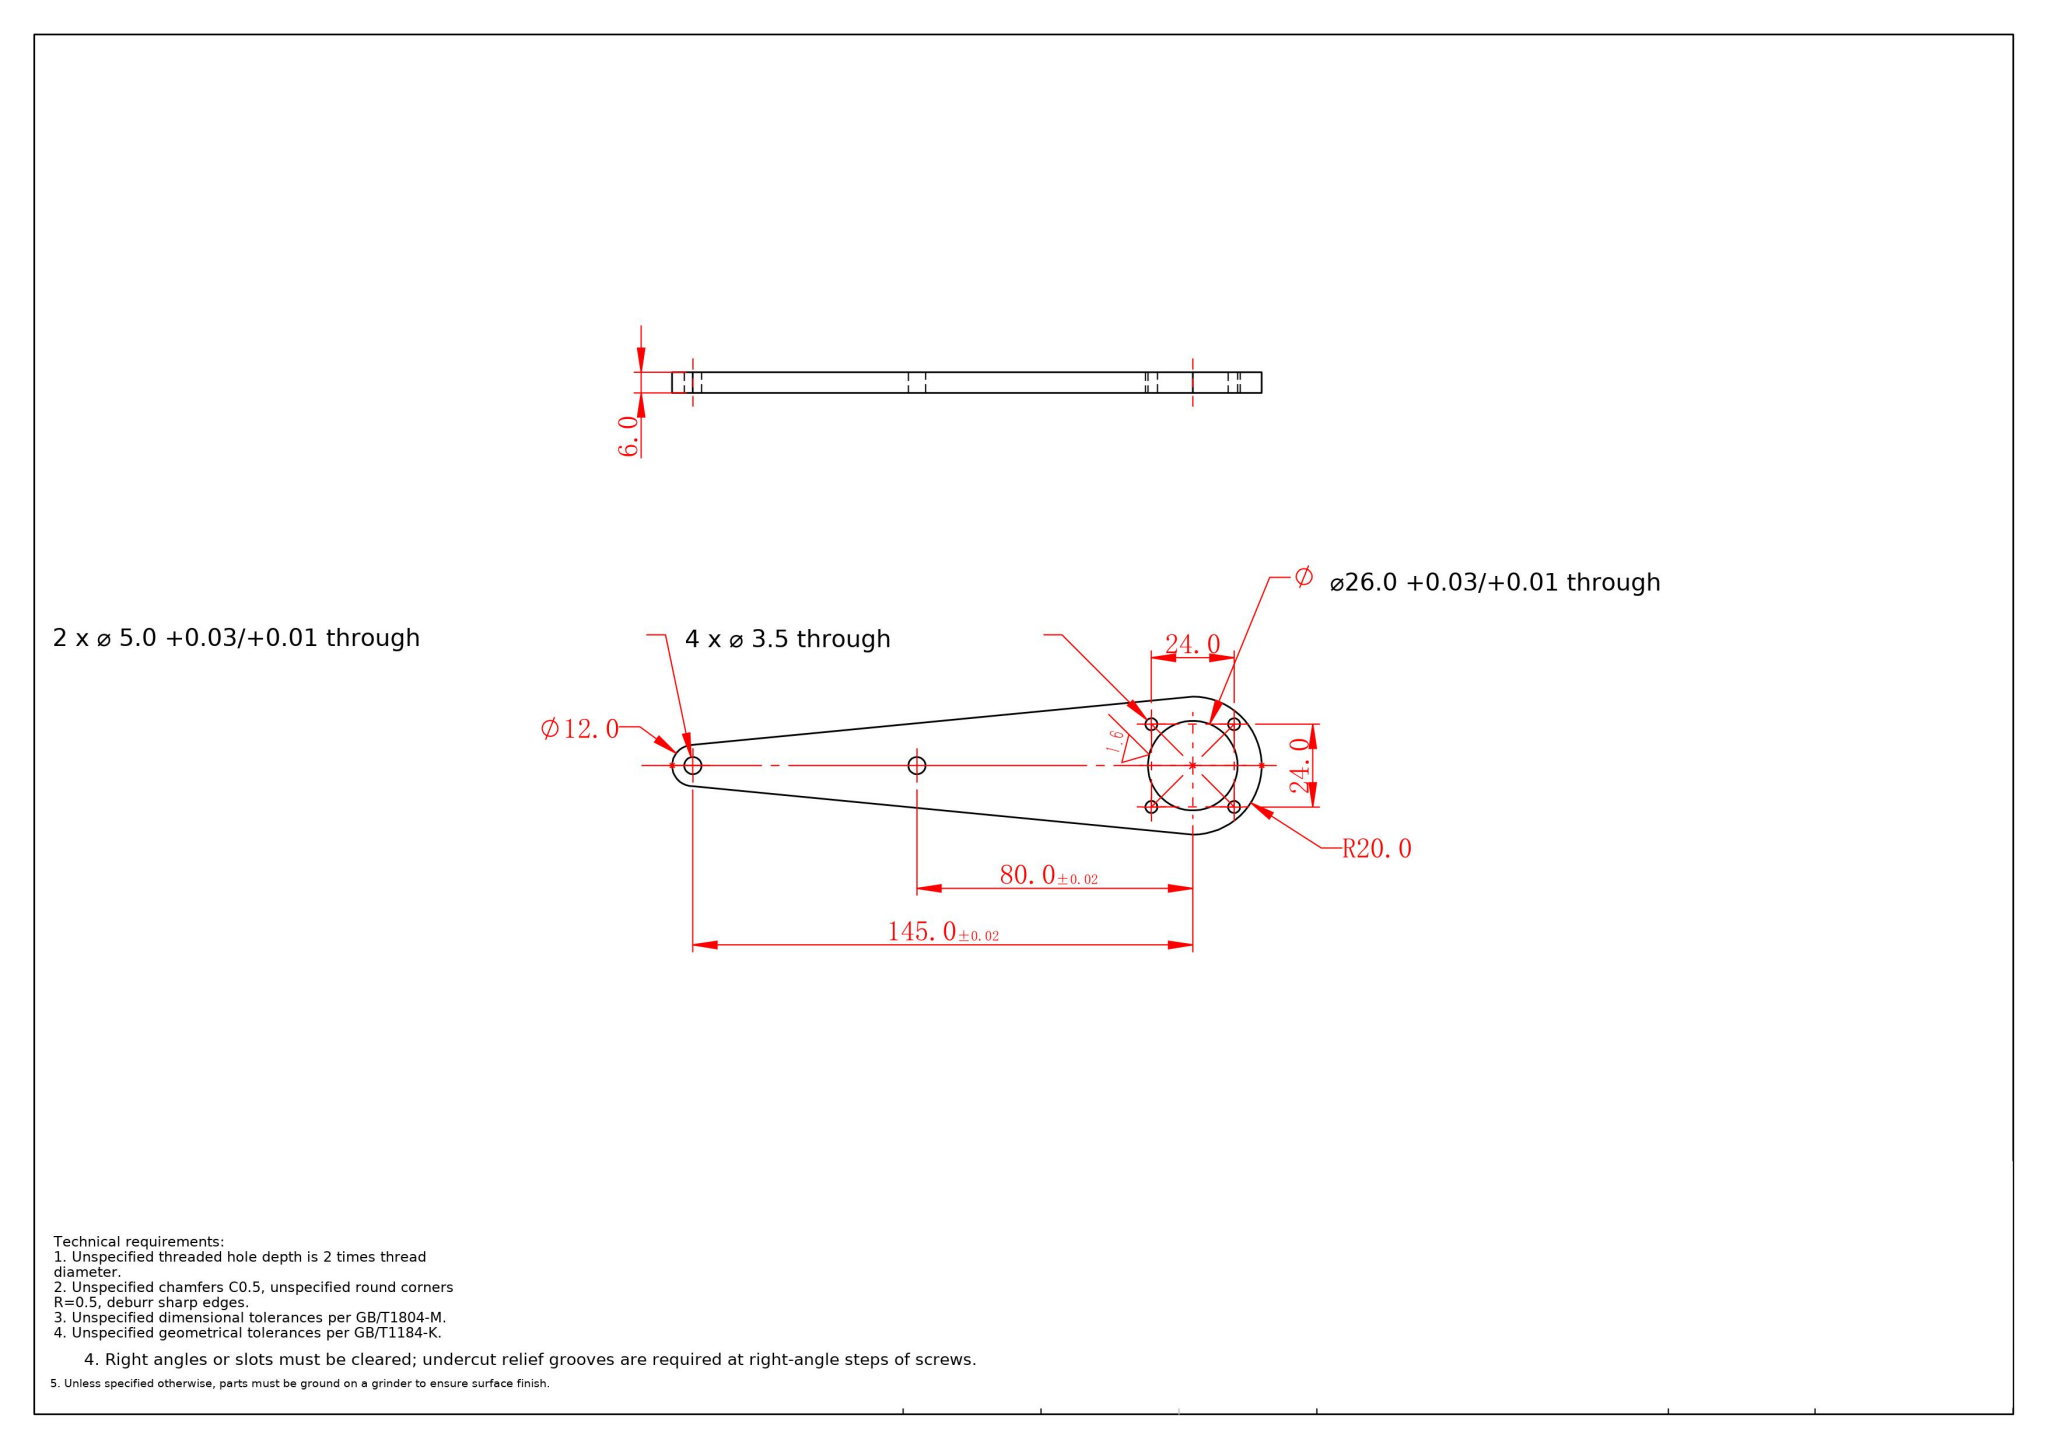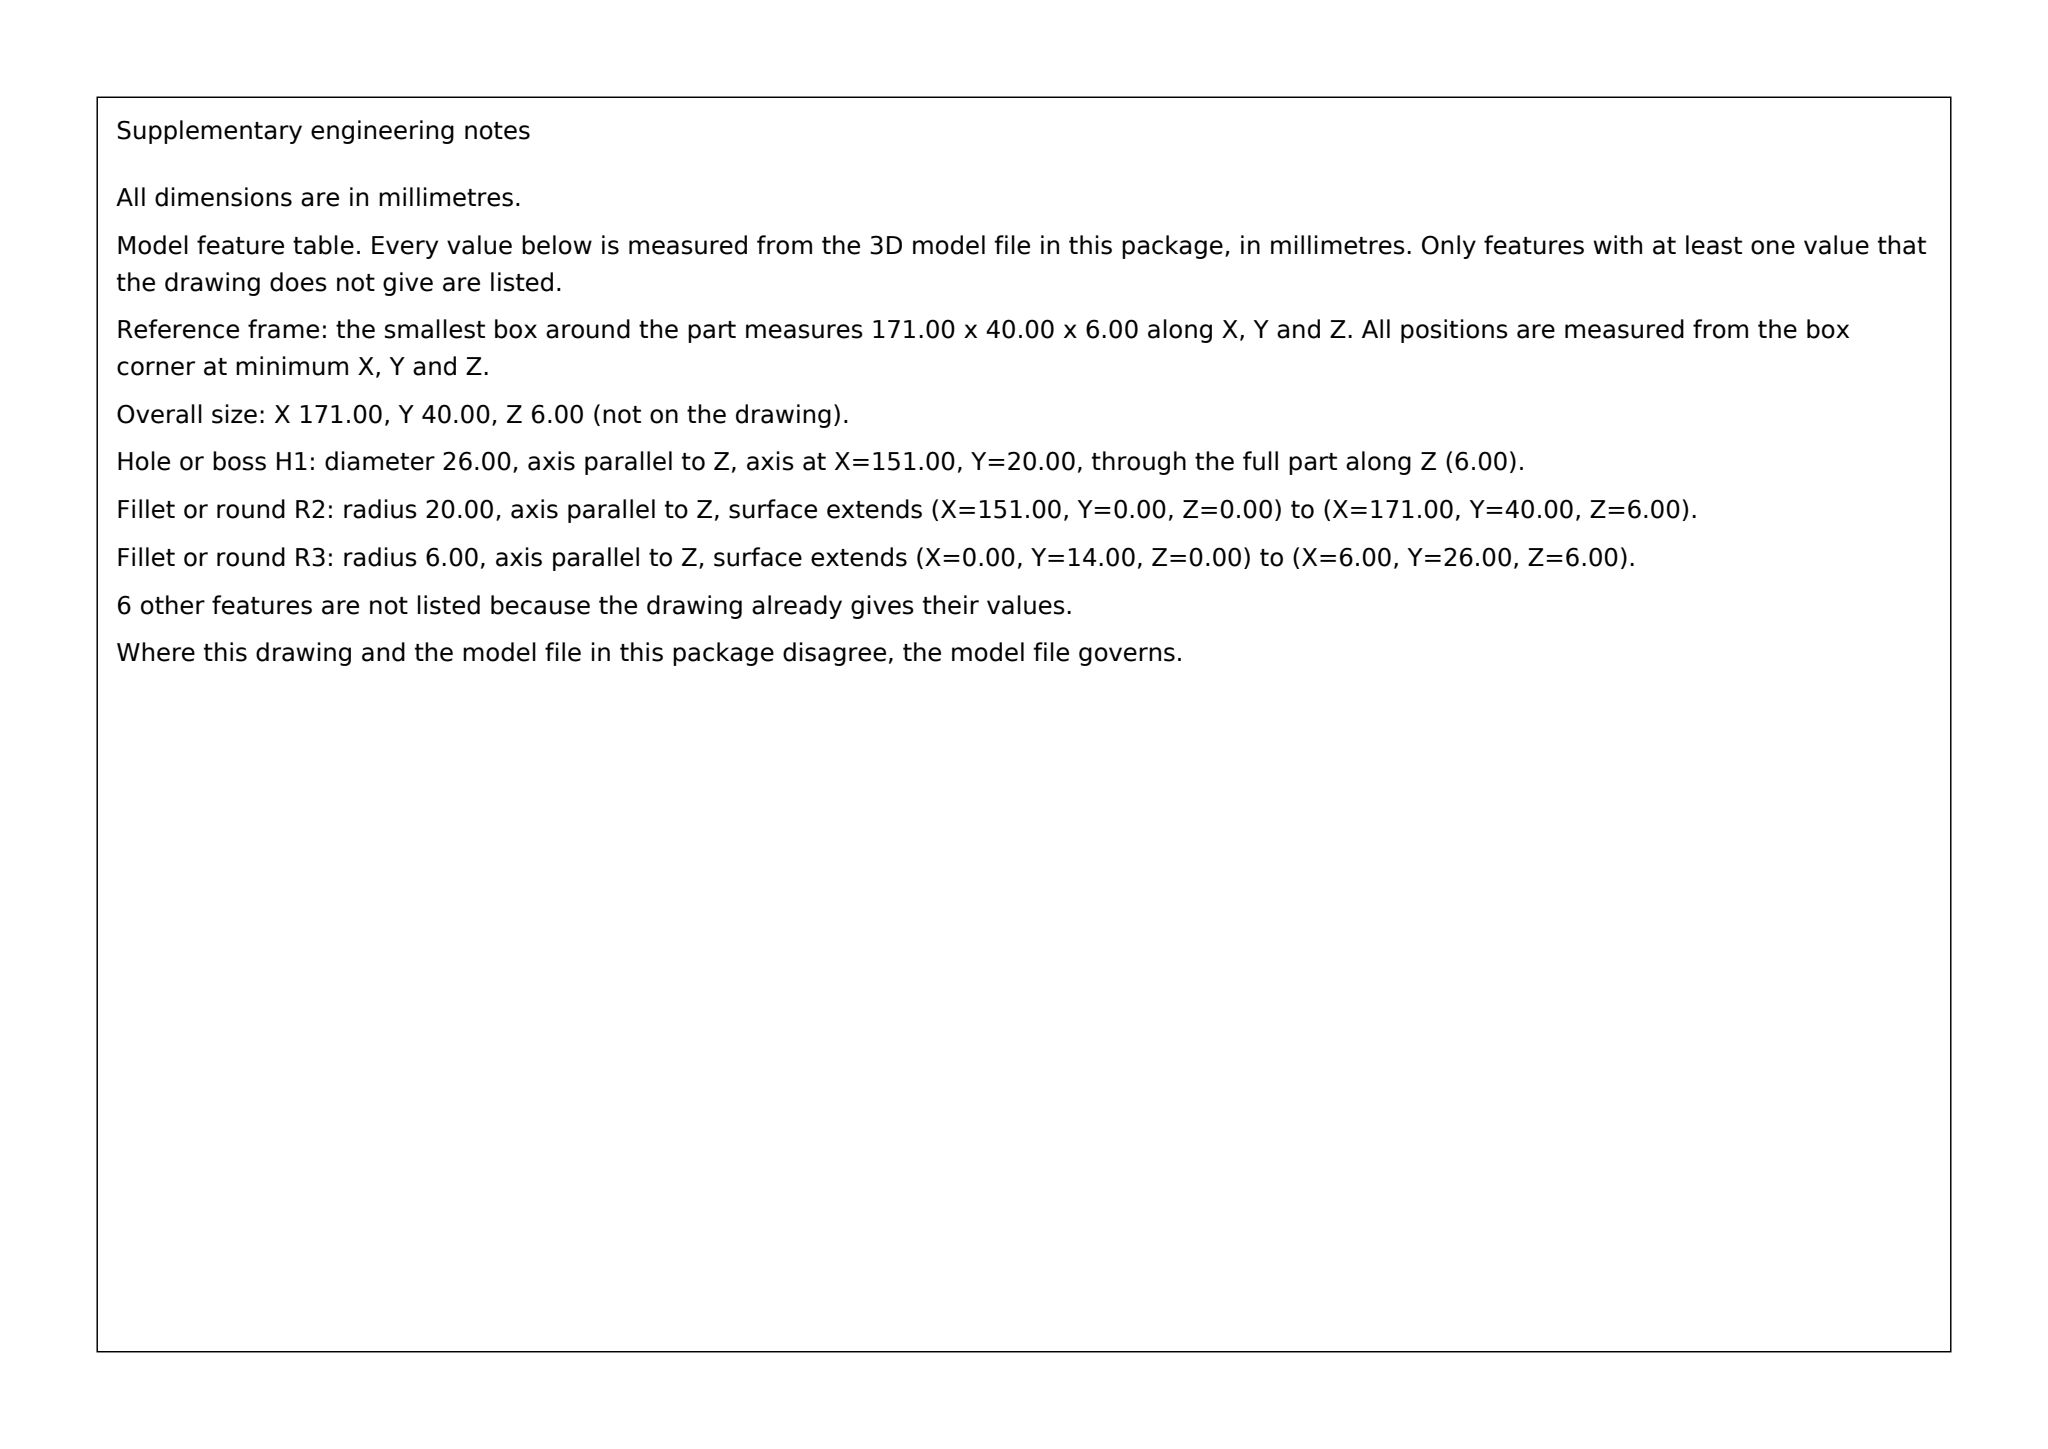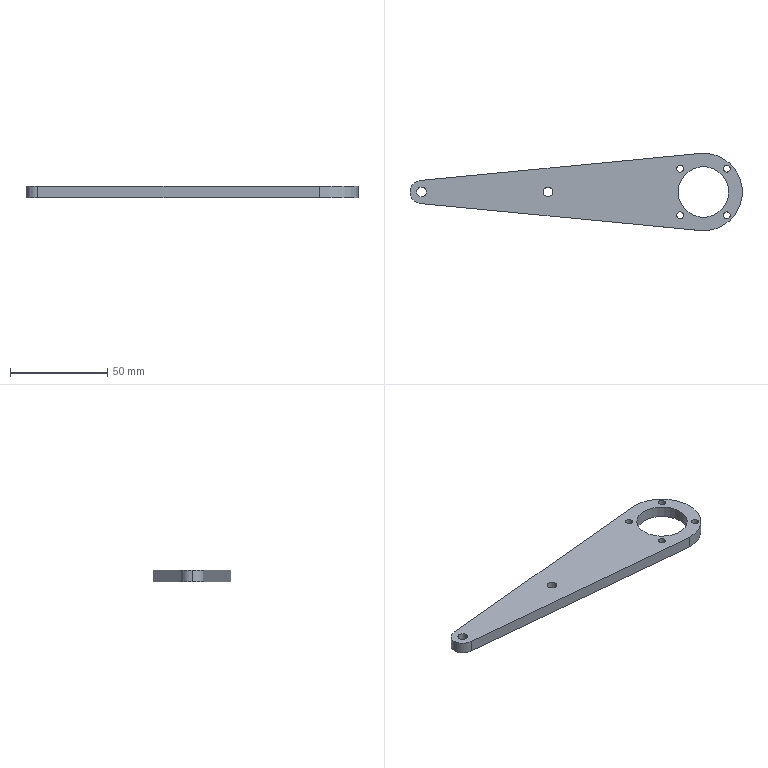Part | SolidWorks | mm | 1 solid | 21 faces | box 171 x 40 x 6 mm | volume 23077 mm3 | cylinder 17 | plane 4 | commonest cylinder face diameters 3.5 x8 5 x4 26 x2 12 x2 40 x1
build123d program:
from build123d import *

# Parameters (mm, degrees)
SKETCH1_R                      = 13
BOSS_EXTRUDE1_DEPTH            = 3
F_3_5_3_5_DIAMETER_HOLE1_D     = 3.5
F_3_5_3_5_DIAMETER_HOLE1_DEPTH = 6
F_5_0_5_DIAMETER_HOLE1_D       = 5


with BuildPart() as part:
    # Sketch1 → Boss-Extrude1 (new, symmetric)
    with BuildSketch(Plane.XY):
        with BuildLine():
            Line((-145, 6), (0, 20))
            ThreePointArc((0, 20), (20, 0), (0, -20))
            Line((0, -20), (-145, -6))
            ThreePointArc((-145, -6), (-151, 0), (-145, 6))
        make_face()
        Circle(SKETCH1_R, mode=Mode.SUBTRACT)
    extrude(amount=BOSS_EXTRUDE1_DEPTH, both=True)

    # 3.5 _3.5_ Diameter Hole1
    with Locations(Plane.XY.offset(3)):
        with Locations((0, 0), (12, -12), (-12, 12), (-12, -12), (12, 12)):
            Hole(F_3_5_3_5_DIAMETER_HOLE1_D / 2, depth=F_3_5_3_5_DIAMETER_HOLE1_DEPTH)

    # 5.0 _5_ Diameter Hole1 (through all)
    with Locations(Plane.XY.offset(3)):
        with Locations((-145, 0), (-80, 0)):
            Hole(F_5_0_5_DIAMETER_HOLE1_D / 2)


solid = part.part
STEP:
#1=CARTESIAN_POINT('',(-147.5,-0.,-3.));
#2=VERTEX_POINT('',#1);
#3=CARTESIAN_POINT('',(-142.5,-0.,-3.));
#4=VERTEX_POINT('',#3);
#5=CARTESIAN_POINT('',(-145.,-0.,-3.));
#6=DIRECTION('',(0.,0.,1.));
#7=DIRECTION('',(1.,0.,0.));
#8=AXIS2_PLACEMENT_3D('',#5,#6,#7);
#9=CIRCLE('',#8,2.5);
#10=EDGE_CURVE('',#2,#4,#9,.T.);
#11=ORIENTED_EDGE('',*,*,#10,.F.);
#12=CARTESIAN_POINT('',(-147.5,-0.,3.));
#13=VERTEX_POINT('',#12);
#14=CARTESIAN_POINT('',(-147.5,-0.,3.));
#15=DIRECTION('',(0.,0.,1.));
#16=VECTOR('',#15,1000.);
#17=LINE('',#14,#16);
#18=EDGE_CURVE('',#2,#13,#17,.T.);
#19=ORIENTED_EDGE('',*,*,#18,.T.);
#20=CARTESIAN_POINT('',(-142.5,-0.,3.));
#21=VERTEX_POINT('',#20);
#22=CARTESIAN_POINT('',(-145.,-0.,3.));
#23=DIRECTION('',(0.,0.,1.));
#24=DIRECTION('',(1.,0.,0.));
#25=AXIS2_PLACEMENT_3D('',#22,#23,#24);
#26=CIRCLE('',#25,2.5);
#27=EDGE_CURVE('',#13,#21,#26,.T.);
#28=ORIENTED_EDGE('',*,*,#27,.T.);
#29=CARTESIAN_POINT('',(-142.5,-0.,3.));
#30=DIRECTION('',(0.,0.,1.));
#31=VECTOR('',#30,1000.);
#32=LINE('',#29,#31);
#33=EDGE_CURVE('',#4,#21,#32,.T.);
#34=ORIENTED_EDGE('',*,*,#33,.F.);
#35=EDGE_LOOP('',(#11,#19,#28,#34));
#36=FACE_OUTER_BOUND('',#35,.T.);
#37=CARTESIAN_POINT('',(-145.,-0.,3.));
#38=DIRECTION('',(0.,0.,1.));
#39=DIRECTION('',(1.,0.,0.));
#40=AXIS2_PLACEMENT_3D('',#37,#38,#39);
#41=CYLINDRICAL_SURFACE('',#40,2.5);
#42=ADVANCED_FACE('',(#36),#41,.F.);
#43=CARTESIAN_POINT('',(-82.5,0.,-3.));
#44=VERTEX_POINT('',#43);
#45=CARTESIAN_POINT('',(-77.5,0.,-3.));
#46=VERTEX_POINT('',#45);
#47=CARTESIAN_POINT('',(-80.,0.,-3.));
#48=DIRECTION('',(0.,0.,1.));
#49=DIRECTION('',(1.,0.,0.));
#50=AXIS2_PLACEMENT_3D('',#47,#48,#49);
#51=CIRCLE('',#50,2.5);
#52=EDGE_CURVE('',#44,#46,#51,.T.);
#53=ORIENTED_EDGE('',*,*,#52,.F.);
#54=CARTESIAN_POINT('',(-82.5,0.,3.));
#55=VERTEX_POINT('',#54);
#56=CARTESIAN_POINT('',(-82.5,0.,3.));
#57=DIRECTION('',(0.,0.,1.));
#58=VECTOR('',#57,1000.);
#59=LINE('',#56,#58);
#60=EDGE_CURVE('',#44,#55,#59,.T.);
#61=ORIENTED_EDGE('',*,*,#60,.T.);
#62=CARTESIAN_POINT('',(-77.5,0.,3.));
#63=VERTEX_POINT('',#62);
#64=CARTESIAN_POINT('',(-80.,0.,3.));
#65=DIRECTION('',(0.,0.,1.));
#66=DIRECTION('',(1.,0.,0.));
#67=AXIS2_PLACEMENT_3D('',#64,#65,#66);
#68=CIRCLE('',#67,2.5);
#69=EDGE_CURVE('',#55,#63,#68,.T.);
#70=ORIENTED_EDGE('',*,*,#69,.T.);
#71=CARTESIAN_POINT('',(-77.5,0.,3.));
#72=DIRECTION('',(0.,0.,1.));
#73=VECTOR('',#72,1000.);
#74=LINE('',#71,#73);
#75=EDGE_CURVE('',#46,#63,#74,.T.);
#76=ORIENTED_EDGE('',*,*,#75,.F.);
#77=EDGE_LOOP('',(#53,#61,#70,#76));
#78=FACE_OUTER_BOUND('',#77,.T.);
#79=CARTESIAN_POINT('',(-80.,0.,3.));
#80=DIRECTION('',(0.,0.,1.));
#81=DIRECTION('',(1.,0.,0.));
#82=AXIS2_PLACEMENT_3D('',#79,#80,#81);
#83=CYLINDRICAL_SURFACE('',#82,2.5);
#84=ADVANCED_FACE('',(#78),#83,.F.);
#85=CARTESIAN_POINT('',(10.25,-12.,-3.));
#86=VERTEX_POINT('',#85);
#87=CARTESIAN_POINT('',(13.75,-12.,-3.));
#88=VERTEX_POINT('',#87);
#89=CARTESIAN_POINT('',(12.,-12.,-3.));
#90=DIRECTION('',(0.,0.,1.));
#91=DIRECTION('',(1.,0.,0.));
#92=AXIS2_PLACEMENT_3D('',#89,#90,#91);
#93=CIRCLE('',#92,1.75);
#94=EDGE_CURVE('',#86,#88,#93,.T.);
#95=ORIENTED_EDGE('',*,*,#94,.F.);
#96=CARTESIAN_POINT('',(10.25,-12.,3.));
#97=VERTEX_POINT('',#96);
#98=CARTESIAN_POINT('',(10.25,-12.,3.));
#99=DIRECTION('',(0.,0.,1.));
#100=VECTOR('',#99,1000.);
#101=LINE('',#98,#100);
#102=EDGE_CURVE('',#86,#97,#101,.T.);
#103=ORIENTED_EDGE('',*,*,#102,.T.);
#104=CARTESIAN_POINT('',(13.75,-12.,3.));
#105=VERTEX_POINT('',#104);
#106=CARTESIAN_POINT('',(12.,-12.,3.));
#107=DIRECTION('',(0.,0.,1.));
#108=DIRECTION('',(1.,0.,0.));
#109=AXIS2_PLACEMENT_3D('',#106,#107,#108);
#110=CIRCLE('',#109,1.75);
#111=EDGE_CURVE('',#97,#105,#110,.T.);
#112=ORIENTED_EDGE('',*,*,#111,.T.);
#113=CARTESIAN_POINT('',(13.75,-12.,3.));
#114=DIRECTION('',(0.,0.,1.));
#115=VECTOR('',#114,1000.);
#116=LINE('',#113,#115);
#117=EDGE_CURVE('',#88,#105,#116,.T.);
#118=ORIENTED_EDGE('',*,*,#117,.F.);
#119=EDGE_LOOP('',(#95,#103,#112,#118));
#120=FACE_OUTER_BOUND('',#119,.T.);
#121=CARTESIAN_POINT('',(12.,-12.,3.));
#122=DIRECTION('',(0.,0.,1.));
#123=DIRECTION('',(1.,0.,0.));
#124=AXIS2_PLACEMENT_3D('',#121,#122,#123);
#125=CYLINDRICAL_SURFACE('',#124,1.75);
#126=ADVANCED_FACE('',(#120),#125,.F.);
#127=CARTESIAN_POINT('',(-13.75,12.,-3.));
#128=VERTEX_POINT('',#127);
#129=CARTESIAN_POINT('',(-10.25,12.,-3.));
#130=VERTEX_POINT('',#129);
#131=CARTESIAN_POINT('',(-12.,12.,-3.));
#132=DIRECTION('',(0.,0.,1.));
#133=DIRECTION('',(1.,0.,0.));
#134=AXIS2_PLACEMENT_3D('',#131,#132,#133);
#135=CIRCLE('',#134,1.75);
#136=EDGE_CURVE('',#128,#130,#135,.T.);
#137=ORIENTED_EDGE('',*,*,#136,.F.);
#138=CARTESIAN_POINT('',(-13.75,12.,3.));
#139=VERTEX_POINT('',#138);
#140=CARTESIAN_POINT('',(-13.75,12.,3.));
#141=DIRECTION('',(0.,0.,1.));
#142=VECTOR('',#141,1000.);
#143=LINE('',#140,#142);
#144=EDGE_CURVE('',#128,#139,#143,.T.);
#145=ORIENTED_EDGE('',*,*,#144,.T.);
#146=CARTESIAN_POINT('',(-10.25,12.,3.));
#147=VERTEX_POINT('',#146);
#148=CARTESIAN_POINT('',(-12.,12.,3.));
#149=DIRECTION('',(0.,0.,1.));
#150=DIRECTION('',(1.,0.,0.));
#151=AXIS2_PLACEMENT_3D('',#148,#149,#150);
#152=CIRCLE('',#151,1.75);
#153=EDGE_CURVE('',#139,#147,#152,.T.);
#154=ORIENTED_EDGE('',*,*,#153,.T.);
#155=CARTESIAN_POINT('',(-10.25,12.,3.));
#156=DIRECTION('',(0.,0.,1.));
#157=VECTOR('',#156,1000.);
#158=LINE('',#155,#157);
#159=EDGE_CURVE('',#130,#147,#158,.T.);
#160=ORIENTED_EDGE('',*,*,#159,.F.);
#161=EDGE_LOOP('',(#137,#145,#154,#160));
#162=FACE_OUTER_BOUND('',#161,.T.);
#163=CARTESIAN_POINT('',(-12.,12.,3.));
#164=DIRECTION('',(0.,0.,1.));
#165=DIRECTION('',(1.,0.,0.));
#166=AXIS2_PLACEMENT_3D('',#163,#164,#165);
#167=CYLINDRICAL_SURFACE('',#166,1.75);
#168=ADVANCED_FACE('',(#162),#167,.F.);
#169=CARTESIAN_POINT('',(-13.75,-12.,-3.));
#170=VERTEX_POINT('',#169);
#171=CARTESIAN_POINT('',(-10.25,-12.,-3.));
#172=VERTEX_POINT('',#171);
#173=CARTESIAN_POINT('',(-12.,-12.,-3.));
#174=DIRECTION('',(0.,0.,1.));
#175=DIRECTION('',(1.,0.,0.));
#176=AXIS2_PLACEMENT_3D('',#173,#174,#175);
#177=CIRCLE('',#176,1.75);
#178=EDGE_CURVE('',#170,#172,#177,.T.);
#179=ORIENTED_EDGE('',*,*,#178,.F.);
#180=CARTESIAN_POINT('',(-13.75,-12.,3.));
#181=VERTEX_POINT('',#180);
#182=CARTESIAN_POINT('',(-13.75,-12.,3.));
#183=DIRECTION('',(0.,0.,1.));
#184=VECTOR('',#183,1000.);
#185=LINE('',#182,#184);
#186=EDGE_CURVE('',#170,#181,#185,.T.);
#187=ORIENTED_EDGE('',*,*,#186,.T.);
#188=CARTESIAN_POINT('',(-10.25,-12.,3.));
#189=VERTEX_POINT('',#188);
#190=CARTESIAN_POINT('',(-12.,-12.,3.));
#191=DIRECTION('',(0.,0.,1.));
#192=DIRECTION('',(1.,0.,0.));
#193=AXIS2_PLACEMENT_3D('',#190,#191,#192);
#194=CIRCLE('',#193,1.75);
#195=EDGE_CURVE('',#181,#189,#194,.T.);
#196=ORIENTED_EDGE('',*,*,#195,.T.);
#197=CARTESIAN_POINT('',(-10.25,-12.,3.));
#198=DIRECTION('',(0.,0.,1.));
#199=VECTOR('',#198,1000.);
#200=LINE('',#197,#199);
#201=EDGE_CURVE('',#172,#189,#200,.T.);
#202=ORIENTED_EDGE('',*,*,#201,.F.);
#203=EDGE_LOOP('',(#179,#187,#196,#202));
#204=FACE_OUTER_BOUND('',#203,.T.);
#205=CARTESIAN_POINT('',(-12.,-12.,3.));
#206=DIRECTION('',(0.,0.,1.));
#207=DIRECTION('',(1.,0.,0.));
#208=AXIS2_PLACEMENT_3D('',#205,#206,#207);
#209=CYLINDRICAL_SURFACE('',#208,1.75);
#210=ADVANCED_FACE('',(#204),#209,.F.);
#211=CARTESIAN_POINT('',(10.25,12.,-3.));
#212=VERTEX_POINT('',#211);
#213=CARTESIAN_POINT('',(13.75,12.,-3.));
#214=VERTEX_POINT('',#213);
#215=CARTESIAN_POINT('',(12.,12.,-3.));
#216=DIRECTION('',(0.,0.,1.));
#217=DIRECTION('',(1.,0.,0.));
#218=AXIS2_PLACEMENT_3D('',#215,#216,#217);
#219=CIRCLE('',#218,1.75);
#220=EDGE_CURVE('',#212,#214,#219,.T.);
#221=ORIENTED_EDGE('',*,*,#220,.F.);
#222=CARTESIAN_POINT('',(10.25,12.,3.));
#223=VERTEX_POINT('',#222);
#224=CARTESIAN_POINT('',(10.25,12.,3.));
#225=DIRECTION('',(0.,0.,1.));
#226=VECTOR('',#225,1000.);
#227=LINE('',#224,#226);
#228=EDGE_CURVE('',#212,#223,#227,.T.);
#229=ORIENTED_EDGE('',*,*,#228,.T.);
#230=CARTESIAN_POINT('',(13.75,12.,3.));
#231=VERTEX_POINT('',#230);
#232=CARTESIAN_POINT('',(12.,12.,3.));
#233=DIRECTION('',(0.,0.,1.));
#234=DIRECTION('',(1.,0.,0.));
#235=AXIS2_PLACEMENT_3D('',#232,#233,#234);
#236=CIRCLE('',#235,1.75);
#237=EDGE_CURVE('',#223,#231,#236,.T.);
#238=ORIENTED_EDGE('',*,*,#237,.T.);
#239=CARTESIAN_POINT('',(13.75,12.,3.));
#240=DIRECTION('',(0.,0.,1.));
#241=VECTOR('',#240,1000.);
#242=LINE('',#239,#241);
#243=EDGE_CURVE('',#214,#231,#242,.T.);
#244=ORIENTED_EDGE('',*,*,#243,.F.);
#245=EDGE_LOOP('',(#221,#229,#238,#244));
#246=FACE_OUTER_BOUND('',#245,.T.);
#247=CARTESIAN_POINT('',(12.,12.,3.));
#248=DIRECTION('',(0.,0.,1.));
#249=DIRECTION('',(1.,0.,0.));
#250=AXIS2_PLACEMENT_3D('',#247,#248,#249);
#251=CYLINDRICAL_SURFACE('',#250,1.75);
#252=ADVANCED_FACE('',(#246),#251,.F.);
#253=CARTESIAN_POINT('',(-13.,0.,3.));
#254=VERTEX_POINT('',#253);
#255=CARTESIAN_POINT('',(13.,0.,3.));
#256=VERTEX_POINT('',#255);
#257=CARTESIAN_POINT('',(0.,0.,3.));
#258=DIRECTION('',(0.,0.,1.));
#259=DIRECTION('',(1.,0.,0.));
#260=AXIS2_PLACEMENT_3D('',#257,#258,#259);
#261=CIRCLE('',#260,13.);
#262=EDGE_CURVE('',#254,#256,#261,.T.);
#263=ORIENTED_EDGE('',*,*,#262,.T.);
#264=CARTESIAN_POINT('',(13.,0.,-3.));
#265=VERTEX_POINT('',#264);
#266=CARTESIAN_POINT('',(13.,0.,3.));
#267=DIRECTION('',(0.,0.,-1.));
#268=VECTOR('',#267,1000.);
#269=LINE('',#266,#268);
#270=EDGE_CURVE('',#256,#265,#269,.T.);
#271=ORIENTED_EDGE('',*,*,#270,.T.);
#272=CARTESIAN_POINT('',(-13.,0.,-3.));
#273=VERTEX_POINT('',#272);
#274=CARTESIAN_POINT('',(0.,0.,-3.));
#275=DIRECTION('',(0.,0.,1.));
#276=DIRECTION('',(1.,0.,0.));
#277=AXIS2_PLACEMENT_3D('',#274,#275,#276);
#278=CIRCLE('',#277,13.);
#279=EDGE_CURVE('',#273,#265,#278,.T.);
#280=ORIENTED_EDGE('',*,*,#279,.F.);
#281=CARTESIAN_POINT('',(-13.,0.,3.));
#282=DIRECTION('',(0.,0.,-1.));
#283=VECTOR('',#282,1000.);
#284=LINE('',#281,#283);
#285=EDGE_CURVE('',#254,#273,#284,.T.);
#286=ORIENTED_EDGE('',*,*,#285,.F.);
#287=EDGE_LOOP('',(#263,#271,#280,#286));
#288=FACE_OUTER_BOUND('',#287,.T.);
#289=CARTESIAN_POINT('',(0.,0.,3.));
#290=DIRECTION('',(0.,0.,-1.));
#291=DIRECTION('',(-1.,0.,0.));
#292=AXIS2_PLACEMENT_3D('',#289,#290,#291);
#293=CYLINDRICAL_SURFACE('',#292,13.);
#294=ADVANCED_FACE('',(#288),#293,.F.);
#295=CARTESIAN_POINT('',(-151.,-0.,3.));
#296=VERTEX_POINT('',#295);
#297=CARTESIAN_POINT('',(-145.,-6.,3.));
#298=VERTEX_POINT('',#297);
#299=CARTESIAN_POINT('',(-145.,-0.,3.));
#300=DIRECTION('',(0.,0.,1.));
#301=DIRECTION('',(1.,0.,0.));
#302=AXIS2_PLACEMENT_3D('',#299,#300,#301);
#303=CIRCLE('',#302,6.);
#304=EDGE_CURVE('',#296,#298,#303,.T.);
#305=ORIENTED_EDGE('',*,*,#304,.F.);
#306=CARTESIAN_POINT('',(-151.,-0.,-3.));
#307=VERTEX_POINT('',#306);
#308=CARTESIAN_POINT('',(-151.,-0.,3.));
#309=DIRECTION('',(0.,0.,-1.));
#310=VECTOR('',#309,1000.);
#311=LINE('',#308,#310);
#312=EDGE_CURVE('',#296,#307,#311,.T.);
#313=ORIENTED_EDGE('',*,*,#312,.T.);
#314=CARTESIAN_POINT('',(-145.,-6.,-3.));
#315=VERTEX_POINT('',#314);
#316=CARTESIAN_POINT('',(-145.,-0.,-3.));
#317=DIRECTION('',(0.,0.,1.));
#318=DIRECTION('',(1.,0.,0.));
#319=AXIS2_PLACEMENT_3D('',#316,#317,#318);
#320=CIRCLE('',#319,6.);
#321=EDGE_CURVE('',#307,#315,#320,.T.);
#322=ORIENTED_EDGE('',*,*,#321,.T.);
#323=CARTESIAN_POINT('',(-145.,-6.,3.));
#324=DIRECTION('',(0.,0.,-1.));
#325=VECTOR('',#324,1000.);
#326=LINE('',#323,#325);
#327=EDGE_CURVE('',#298,#315,#326,.T.);
#328=ORIENTED_EDGE('',*,*,#327,.F.);
#329=EDGE_LOOP('',(#305,#313,#322,#328));
#330=FACE_OUTER_BOUND('',#329,.T.);
#331=CARTESIAN_POINT('',(-145.,-0.,3.));
#332=DIRECTION('',(0.,0.,-1.));
#333=DIRECTION('',(-1.,0.,0.));
#334=AXIS2_PLACEMENT_3D('',#331,#332,#333);
#335=CYLINDRICAL_SURFACE('',#334,6.);
#336=ADVANCED_FACE('',(#330),#335,.T.);
#337=CARTESIAN_POINT('',(-145.,-0.,3.));
#338=DIRECTION('',(0.,0.,1.));
#339=DIRECTION('',(1.,0.,0.));
#340=AXIS2_PLACEMENT_3D('',#337,#338,#339);
#341=CIRCLE('',#340,2.5);
#342=EDGE_CURVE('',#21,#13,#341,.T.);
#343=ORIENTED_EDGE('',*,*,#342,.F.);
#344=ORIENTED_EDGE('',*,*,#27,.F.);
#345=EDGE_LOOP('',(#343,#344));
#346=FACE_BOUND('',#345,.T.);
#347=CARTESIAN_POINT('',(-80.,0.,3.));
#348=DIRECTION('',(0.,0.,1.));
#349=DIRECTION('',(1.,0.,0.));
#350=AXIS2_PLACEMENT_3D('',#347,#348,#349);
#351=CIRCLE('',#350,2.5);
#352=EDGE_CURVE('',#63,#55,#351,.T.);
#353=ORIENTED_EDGE('',*,*,#352,.F.);
#354=ORIENTED_EDGE('',*,*,#69,.F.);
#355=EDGE_LOOP('',(#353,#354));
#356=FACE_BOUND('',#355,.T.);
#357=CARTESIAN_POINT('',(12.,-12.,3.));
#358=DIRECTION('',(0.,0.,1.));
#359=DIRECTION('',(1.,0.,0.));
#360=AXIS2_PLACEMENT_3D('',#357,#358,#359);
#361=CIRCLE('',#360,1.75);
#362=EDGE_CURVE('',#105,#97,#361,.T.);
#363=ORIENTED_EDGE('',*,*,#362,.F.);
#364=ORIENTED_EDGE('',*,*,#111,.F.);
#365=EDGE_LOOP('',(#363,#364));
#366=FACE_BOUND('',#365,.T.);
#367=CARTESIAN_POINT('',(-12.,12.,3.));
#368=DIRECTION('',(0.,0.,1.));
#369=DIRECTION('',(1.,0.,0.));
#370=AXIS2_PLACEMENT_3D('',#367,#368,#369);
#371=CIRCLE('',#370,1.75);
#372=EDGE_CURVE('',#147,#139,#371,.T.);
#373=ORIENTED_EDGE('',*,*,#372,.F.);
#374=ORIENTED_EDGE('',*,*,#153,.F.);
#375=EDGE_LOOP('',(#373,#374));
#376=FACE_BOUND('',#375,.T.);
#377=CARTESIAN_POINT('',(-12.,-12.,3.));
#378=DIRECTION('',(0.,0.,1.));
#379=DIRECTION('',(1.,0.,0.));
#380=AXIS2_PLACEMENT_3D('',#377,#378,#379);
#381=CIRCLE('',#380,1.75);
#382=EDGE_CURVE('',#189,#181,#381,.T.);
#383=ORIENTED_EDGE('',*,*,#382,.F.);
#384=ORIENTED_EDGE('',*,*,#195,.F.);
#385=EDGE_LOOP('',(#383,#384));
#386=FACE_BOUND('',#385,.T.);
#387=CARTESIAN_POINT('',(12.,12.,3.));
#388=DIRECTION('',(0.,0.,1.));
#389=DIRECTION('',(1.,0.,0.));
#390=AXIS2_PLACEMENT_3D('',#387,#388,#389);
#391=CIRCLE('',#390,1.75);
#392=EDGE_CURVE('',#231,#223,#391,.T.);
#393=ORIENTED_EDGE('',*,*,#392,.F.);
#394=ORIENTED_EDGE('',*,*,#237,.F.);
#395=EDGE_LOOP('',(#393,#394));
#396=FACE_BOUND('',#395,.T.);
#397=CARTESIAN_POINT('',(0.,-20.,3.));
#398=VERTEX_POINT('',#397);
#399=CARTESIAN_POINT('',(0.,20.,3.));
#400=VERTEX_POINT('',#399);
#401=CARTESIAN_POINT('',(0.,0.,3.));
#402=DIRECTION('',(0.,0.,1.));
#403=DIRECTION('',(1.,0.,0.));
#404=AXIS2_PLACEMENT_3D('',#401,#402,#403);
#405=CIRCLE('',#404,20.);
#406=EDGE_CURVE('',#398,#400,#405,.T.);
#407=ORIENTED_EDGE('',*,*,#406,.T.);
#408=CARTESIAN_POINT('',(-145.,6.,3.));
#409=VERTEX_POINT('',#408);
#410=CARTESIAN_POINT('',(-145.,6.,3.));
#411=DIRECTION('',(-0.9954,-0.0961,0.));
#412=VECTOR('',#411,1000.);
#413=LINE('',#410,#412);
#414=EDGE_CURVE('',#400,#409,#413,.T.);
#415=ORIENTED_EDGE('',*,*,#414,.T.);
#416=CARTESIAN_POINT('',(-145.,-0.,3.));
#417=DIRECTION('',(0.,0.,1.));
#418=DIRECTION('',(1.,0.,0.));
#419=AXIS2_PLACEMENT_3D('',#416,#417,#418);
#420=CIRCLE('',#419,6.);
#421=EDGE_CURVE('',#409,#296,#420,.T.);
#422=ORIENTED_EDGE('',*,*,#421,.T.);
#423=ORIENTED_EDGE('',*,*,#304,.T.);
#424=CARTESIAN_POINT('',(-145.,-6.,3.));
#425=DIRECTION('',(0.9954,-0.0961,0.));
#426=VECTOR('',#425,1000.);
#427=LINE('',#424,#426);
#428=EDGE_CURVE('',#298,#398,#427,.T.);
#429=ORIENTED_EDGE('',*,*,#428,.T.);
#430=EDGE_LOOP('',(#407,#415,#422,#423,#429));
#431=FACE_OUTER_BOUND('',#430,.T.);
#432=ORIENTED_EDGE('',*,*,#262,.F.);
#433=CARTESIAN_POINT('',(0.,0.,3.));
#434=DIRECTION('',(0.,0.,1.));
#435=DIRECTION('',(1.,0.,0.));
#436=AXIS2_PLACEMENT_3D('',#433,#434,#435);
#437=CIRCLE('',#436,13.);
#438=EDGE_CURVE('',#256,#254,#437,.T.);
#439=ORIENTED_EDGE('',*,*,#438,.F.);
#440=EDGE_LOOP('',(#432,#439));
#441=FACE_BOUND('',#440,.T.);
#442=CARTESIAN_POINT('',(0.,0.,3.));
#443=DIRECTION('',(0.,0.,1.));
#444=DIRECTION('',(1.,0.,0.));
#445=AXIS2_PLACEMENT_3D('',#442,#443,#444);
#446=PLANE('',#445);
#447=ADVANCED_FACE('',(#346,#356,#366,#376,#386,#396,#431,#441),#446,.T.);
#448=CARTESIAN_POINT('',(-145.,-0.,-3.));
#449=DIRECTION('',(0.,0.,1.));
#450=DIRECTION('',(1.,0.,0.));
#451=AXIS2_PLACEMENT_3D('',#448,#449,#450);
#452=CIRCLE('',#451,2.5);
#453=EDGE_CURVE('',#4,#2,#452,.T.);
#454=ORIENTED_EDGE('',*,*,#453,.T.);
#455=ORIENTED_EDGE('',*,*,#10,.T.);
#456=EDGE_LOOP('',(#454,#455));
#457=FACE_BOUND('',#456,.T.);
#458=CARTESIAN_POINT('',(-80.,0.,-3.));
#459=DIRECTION('',(0.,0.,1.));
#460=DIRECTION('',(1.,0.,0.));
#461=AXIS2_PLACEMENT_3D('',#458,#459,#460);
#462=CIRCLE('',#461,2.5);
#463=EDGE_CURVE('',#46,#44,#462,.T.);
#464=ORIENTED_EDGE('',*,*,#463,.T.);
#465=ORIENTED_EDGE('',*,*,#52,.T.);
#466=EDGE_LOOP('',(#464,#465));
#467=FACE_BOUND('',#466,.T.);
#468=CARTESIAN_POINT('',(12.,-12.,-3.));
#469=DIRECTION('',(0.,0.,1.));
#470=DIRECTION('',(1.,0.,0.));
#471=AXIS2_PLACEMENT_3D('',#468,#469,#470);
#472=CIRCLE('',#471,1.75);
#473=EDGE_CURVE('',#88,#86,#472,.T.);
#474=ORIENTED_EDGE('',*,*,#473,.T.);
#475=ORIENTED_EDGE('',*,*,#94,.T.);
#476=EDGE_LOOP('',(#474,#475));
#477=FACE_BOUND('',#476,.T.);
#478=CARTESIAN_POINT('',(-12.,12.,-3.));
#479=DIRECTION('',(0.,0.,1.));
#480=DIRECTION('',(1.,0.,0.));
#481=AXIS2_PLACEMENT_3D('',#478,#479,#480);
#482=CIRCLE('',#481,1.75);
#483=EDGE_CURVE('',#130,#128,#482,.T.);
#484=ORIENTED_EDGE('',*,*,#483,.T.);
#485=ORIENTED_EDGE('',*,*,#136,.T.);
#486=EDGE_LOOP('',(#484,#485));
#487=FACE_BOUND('',#486,.T.);
#488=CARTESIAN_POINT('',(-12.,-12.,-3.));
#489=DIRECTION('',(0.,0.,1.));
#490=DIRECTION('',(1.,0.,0.));
#491=AXIS2_PLACEMENT_3D('',#488,#489,#490);
#492=CIRCLE('',#491,1.75);
#493=EDGE_CURVE('',#172,#170,#492,.T.);
#494=ORIENTED_EDGE('',*,*,#493,.T.);
#495=ORIENTED_EDGE('',*,*,#178,.T.);
#496=EDGE_LOOP('',(#494,#495));
#497=FACE_BOUND('',#496,.T.);
#498=CARTESIAN_POINT('',(12.,12.,-3.));
#499=DIRECTION('',(0.,0.,1.));
#500=DIRECTION('',(1.,0.,0.));
#501=AXIS2_PLACEMENT_3D('',#498,#499,#500);
#502=CIRCLE('',#501,1.75);
#503=EDGE_CURVE('',#214,#212,#502,.T.);
#504=ORIENTED_EDGE('',*,*,#503,.T.);
#505=ORIENTED_EDGE('',*,*,#220,.T.);
#506=EDGE_LOOP('',(#504,#505));
#507=FACE_BOUND('',#506,.T.);
#508=CARTESIAN_POINT('',(0.,-20.,-3.));
#509=VERTEX_POINT('',#508);
#510=CARTESIAN_POINT('',(0.,20.,-3.));
#511=VERTEX_POINT('',#510);
#512=CARTESIAN_POINT('',(0.,0.,-3.));
#513=DIRECTION('',(0.,0.,1.));
#514=DIRECTION('',(1.,0.,0.));
#515=AXIS2_PLACEMENT_3D('',#512,#513,#514);
#516=CIRCLE('',#515,20.);
#517=EDGE_CURVE('',#509,#511,#516,.T.);
#518=ORIENTED_EDGE('',*,*,#517,.F.);
#519=CARTESIAN_POINT('',(-145.,-6.,-3.));
#520=DIRECTION('',(0.9954,-0.0961,0.));
#521=VECTOR('',#520,1000.);
#522=LINE('',#519,#521);
#523=EDGE_CURVE('',#315,#509,#522,.T.);
#524=ORIENTED_EDGE('',*,*,#523,.F.);
#525=ORIENTED_EDGE('',*,*,#321,.F.);
#526=CARTESIAN_POINT('',(-145.,6.,-3.));
#527=VERTEX_POINT('',#526);
#528=CARTESIAN_POINT('',(-145.,-0.,-3.));
#529=DIRECTION('',(0.,0.,1.));
#530=DIRECTION('',(1.,0.,0.));
#531=AXIS2_PLACEMENT_3D('',#528,#529,#530);
#532=CIRCLE('',#531,6.);
#533=EDGE_CURVE('',#527,#307,#532,.T.);
#534=ORIENTED_EDGE('',*,*,#533,.F.);
#535=CARTESIAN_POINT('',(-145.,6.,-3.));
#536=DIRECTION('',(-0.9954,-0.0961,0.));
#537=VECTOR('',#536,1000.);
#538=LINE('',#535,#537);
#539=EDGE_CURVE('',#511,#527,#538,.T.);
#540=ORIENTED_EDGE('',*,*,#539,.F.);
#541=EDGE_LOOP('',(#518,#524,#525,#534,#540));
#542=FACE_OUTER_BOUND('',#541,.T.);
#543=ORIENTED_EDGE('',*,*,#279,.T.);
#544=CARTESIAN_POINT('',(0.,0.,-3.));
#545=DIRECTION('',(0.,0.,1.));
#546=DIRECTION('',(1.,0.,0.));
#547=AXIS2_PLACEMENT_3D('',#544,#545,#546);
#548=CIRCLE('',#547,13.);
#549=EDGE_CURVE('',#265,#273,#548,.T.);
#550=ORIENTED_EDGE('',*,*,#549,.T.);
#551=EDGE_LOOP('',(#543,#550));
#552=FACE_BOUND('',#551,.T.);
#553=CARTESIAN_POINT('',(0.,0.,-3.));
#554=DIRECTION('',(0.,0.,1.));
#555=DIRECTION('',(1.,0.,0.));
#556=AXIS2_PLACEMENT_3D('',#553,#554,#555);
#557=PLANE('',#556);
#558=ADVANCED_FACE('',(#457,#467,#477,#487,#497,#507,#542,#552),#557,.F.);
#559=ORIENTED_EDGE('',*,*,#517,.T.);
#560=CARTESIAN_POINT('',(0.,20.,3.));
#561=DIRECTION('',(0.,0.,-1.));
#562=VECTOR('',#561,1000.);
#563=LINE('',#560,#562);
#564=EDGE_CURVE('',#400,#511,#563,.T.);
#565=ORIENTED_EDGE('',*,*,#564,.F.);
#566=ORIENTED_EDGE('',*,*,#406,.F.);
#567=CARTESIAN_POINT('',(0.,-20.,3.));
#568=DIRECTION('',(0.,0.,-1.));
#569=VECTOR('',#568,1000.);
#570=LINE('',#567,#569);
#571=EDGE_CURVE('',#398,#509,#570,.T.);
#572=ORIENTED_EDGE('',*,*,#571,.T.);
#573=EDGE_LOOP('',(#559,#565,#566,#572));
#574=FACE_OUTER_BOUND('',#573,.T.);
#575=CARTESIAN_POINT('',(0.,0.,3.));
#576=DIRECTION('',(0.,0.,-1.));
#577=DIRECTION('',(-1.,0.,0.));
#578=AXIS2_PLACEMENT_3D('',#575,#576,#577);
#579=CYLINDRICAL_SURFACE('',#578,20.);
#580=ADVANCED_FACE('',(#574),#579,.T.);
#581=ORIENTED_EDGE('',*,*,#539,.T.);
#582=CARTESIAN_POINT('',(-145.,6.,3.));
#583=DIRECTION('',(0.,0.,-1.));
#584=VECTOR('',#583,1000.);
#585=LINE('',#582,#584);
#586=EDGE_CURVE('',#409,#527,#585,.T.);
#587=ORIENTED_EDGE('',*,*,#586,.F.);
#588=ORIENTED_EDGE('',*,*,#414,.F.);
#589=ORIENTED_EDGE('',*,*,#564,.T.);
#590=EDGE_LOOP('',(#581,#587,#588,#589));
#591=FACE_OUTER_BOUND('',#590,.T.);
#592=CARTESIAN_POINT('',(-145.,6.,3.));
#593=DIRECTION('',(0.0961,-0.9954,0.));
#594=DIRECTION('',(0.9954,0.0961,0.));
#595=AXIS2_PLACEMENT_3D('',#592,#593,#594);
#596=PLANE('',#595);
#597=ADVANCED_FACE('',(#591),#596,.F.);
#598=ORIENTED_EDGE('',*,*,#312,.F.);
#599=ORIENTED_EDGE('',*,*,#421,.F.);
#600=ORIENTED_EDGE('',*,*,#586,.T.);
#601=ORIENTED_EDGE('',*,*,#533,.T.);
#602=EDGE_LOOP('',(#598,#599,#600,#601));
#603=FACE_OUTER_BOUND('',#602,.T.);
#604=CARTESIAN_POINT('',(-145.,-0.,3.));
#605=DIRECTION('',(0.,0.,-1.));
#606=DIRECTION('',(-1.,0.,0.));
#607=AXIS2_PLACEMENT_3D('',#604,#605,#606);
#608=CYLINDRICAL_SURFACE('',#607,6.);
#609=ADVANCED_FACE('',(#603),#608,.T.);
#610=ORIENTED_EDGE('',*,*,#523,.T.);
#611=ORIENTED_EDGE('',*,*,#571,.F.);
#612=ORIENTED_EDGE('',*,*,#428,.F.);
#613=ORIENTED_EDGE('',*,*,#327,.T.);
#614=EDGE_LOOP('',(#610,#611,#612,#613));
#615=FACE_OUTER_BOUND('',#614,.T.);
#616=CARTESIAN_POINT('',(-145.,-6.,3.));
#617=DIRECTION('',(0.0961,0.9954,0.));
#618=DIRECTION('',(-0.9954,0.0961,0.));
#619=AXIS2_PLACEMENT_3D('',#616,#617,#618);
#620=PLANE('',#619);
#621=ADVANCED_FACE('',(#615),#620,.F.);
#622=ORIENTED_EDGE('',*,*,#270,.F.);
#623=ORIENTED_EDGE('',*,*,#438,.T.);
#624=ORIENTED_EDGE('',*,*,#285,.T.);
#625=ORIENTED_EDGE('',*,*,#549,.F.);
#626=EDGE_LOOP('',(#622,#623,#624,#625));
#627=FACE_OUTER_BOUND('',#626,.T.);
#628=CARTESIAN_POINT('',(0.,0.,3.));
#629=DIRECTION('',(0.,0.,-1.));
#630=DIRECTION('',(-1.,0.,0.));
#631=AXIS2_PLACEMENT_3D('',#628,#629,#630);
#632=CYLINDRICAL_SURFACE('',#631,13.);
#633=ADVANCED_FACE('',(#627),#632,.F.);
#634=ORIENTED_EDGE('',*,*,#228,.F.);
#635=ORIENTED_EDGE('',*,*,#503,.F.);
#636=ORIENTED_EDGE('',*,*,#243,.T.);
#637=ORIENTED_EDGE('',*,*,#392,.T.);
#638=EDGE_LOOP('',(#634,#635,#636,#637));
#639=FACE_OUTER_BOUND('',#638,.T.);
#640=CARTESIAN_POINT('',(12.,12.,3.));
#641=DIRECTION('',(0.,0.,1.));
#642=DIRECTION('',(1.,0.,0.));
#643=AXIS2_PLACEMENT_3D('',#640,#641,#642);
#644=CYLINDRICAL_SURFACE('',#643,1.75);
#645=ADVANCED_FACE('',(#639),#644,.F.);
#646=ORIENTED_EDGE('',*,*,#186,.F.);
#647=ORIENTED_EDGE('',*,*,#493,.F.);
#648=ORIENTED_EDGE('',*,*,#201,.T.);
#649=ORIENTED_EDGE('',*,*,#382,.T.);
#650=EDGE_LOOP('',(#646,#647,#648,#649));
#651=FACE_OUTER_BOUND('',#650,.T.);
#652=CARTESIAN_POINT('',(-12.,-12.,3.));
#653=DIRECTION('',(0.,0.,1.));
#654=DIRECTION('',(1.,0.,0.));
#655=AXIS2_PLACEMENT_3D('',#652,#653,#654);
#656=CYLINDRICAL_SURFACE('',#655,1.75);
#657=ADVANCED_FACE('',(#651),#656,.F.);
#658=ORIENTED_EDGE('',*,*,#144,.F.);
#659=ORIENTED_EDGE('',*,*,#483,.F.);
#660=ORIENTED_EDGE('',*,*,#159,.T.);
#661=ORIENTED_EDGE('',*,*,#372,.T.);
#662=EDGE_LOOP('',(#658,#659,#660,#661));
#663=FACE_OUTER_BOUND('',#662,.T.);
#664=CARTESIAN_POINT('',(-12.,12.,3.));
#665=DIRECTION('',(0.,0.,1.));
#666=DIRECTION('',(1.,0.,0.));
#667=AXIS2_PLACEMENT_3D('',#664,#665,#666);
#668=CYLINDRICAL_SURFACE('',#667,1.75);
#669=ADVANCED_FACE('',(#663),#668,.F.);
#670=ORIENTED_EDGE('',*,*,#102,.F.);
#671=ORIENTED_EDGE('',*,*,#473,.F.);
#672=ORIENTED_EDGE('',*,*,#117,.T.);
#673=ORIENTED_EDGE('',*,*,#362,.T.);
#674=EDGE_LOOP('',(#670,#671,#672,#673));
#675=FACE_OUTER_BOUND('',#674,.T.);
#676=CARTESIAN_POINT('',(12.,-12.,3.));
#677=DIRECTION('',(0.,0.,1.));
#678=DIRECTION('',(1.,0.,0.));
#679=AXIS2_PLACEMENT_3D('',#676,#677,#678);
#680=CYLINDRICAL_SURFACE('',#679,1.75);
#681=ADVANCED_FACE('',(#675),#680,.F.);
#682=ORIENTED_EDGE('',*,*,#60,.F.);
#683=ORIENTED_EDGE('',*,*,#463,.F.);
#684=ORIENTED_EDGE('',*,*,#75,.T.);
#685=ORIENTED_EDGE('',*,*,#352,.T.);
#686=EDGE_LOOP('',(#682,#683,#684,#685));
#687=FACE_OUTER_BOUND('',#686,.T.);
#688=CARTESIAN_POINT('',(-80.,0.,3.));
#689=DIRECTION('',(0.,0.,1.));
#690=DIRECTION('',(1.,0.,0.));
#691=AXIS2_PLACEMENT_3D('',#688,#689,#690);
#692=CYLINDRICAL_SURFACE('',#691,2.5);
#693=ADVANCED_FACE('',(#687),#692,.F.);
#694=ORIENTED_EDGE('',*,*,#18,.F.);
#695=ORIENTED_EDGE('',*,*,#453,.F.);
#696=ORIENTED_EDGE('',*,*,#33,.T.);
#697=ORIENTED_EDGE('',*,*,#342,.T.);
#698=EDGE_LOOP('',(#694,#695,#696,#697));
#699=FACE_OUTER_BOUND('',#698,.T.);
#700=CARTESIAN_POINT('',(-145.,-0.,3.));
#701=DIRECTION('',(0.,0.,1.));
#702=DIRECTION('',(1.,0.,0.));
#703=AXIS2_PLACEMENT_3D('',#700,#701,#702);
#704=CYLINDRICAL_SURFACE('',#703,2.5);
#705=ADVANCED_FACE('',(#699),#704,.F.);
#706=CLOSED_SHELL('',(#42,#84,#126,#168,#210,#252,#294,#336,#447,#558,#580,#597,#609,#621,#633,#645,#657,#669,#681,#693,#705));
#707=MANIFOLD_SOLID_BREP('',#706);
#708=CARTESIAN_POINT('',(0.,0.,0.));
#709=DIRECTION('',(0.,0.,1.));
#710=DIRECTION('',(1.,0.,0.));
#711=AXIS2_PLACEMENT_3D('',#708,#709,#710);
#712=(LENGTH_UNIT()NAMED_UNIT(*)SI_UNIT(.MILLI.,.METRE.));
#713=UNCERTAINTY_MEASURE_WITH_UNIT(LENGTH_MEASURE(0.00001),#712,'','');
#714=(NAMED_UNIT(*)PLANE_ANGLE_UNIT()SI_UNIT($,.RADIAN.));
#715=(NAMED_UNIT(*)SI_UNIT($,.STERADIAN.)SOLID_ANGLE_UNIT());
#716=(GEOMETRIC_REPRESENTATION_CONTEXT(3)GLOBAL_UNCERTAINTY_ASSIGNED_CONTEXT((#713))GLOBAL_UNIT_ASSIGNED_CONTEXT((#712,#714,#715))REPRESENTATION_CONTEXT('',''));
#717=ADVANCED_BREP_SHAPE_REPRESENTATION('',(#707,#711),#716);